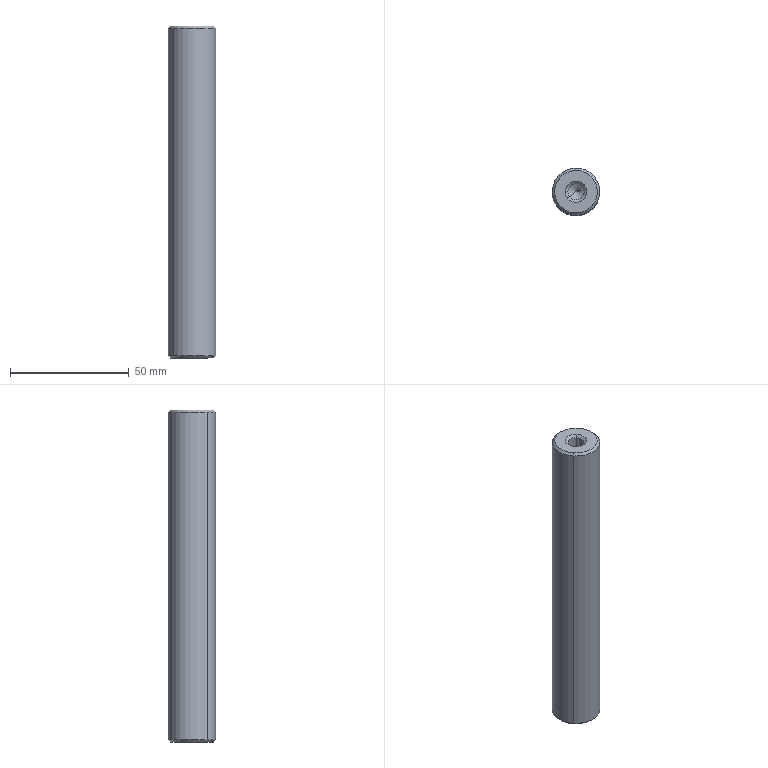Component | SolidWorks | Column-1 | 1 solid | 20 faces | box 20 x 20 x 140 mm | volume 42231 mm3 | cone 12 | cylinder 6 | plane 2 | commonest cylinder face diameters 6.8 x4 20 x2
STEP:
#1=COLOUR_RGB('',0.7922,0.8196,0.9333);
#2=FILL_AREA_STYLE_COLOUR('',#1);
#3=FILL_AREA_STYLE('',(#2));
#4=SURFACE_STYLE_FILL_AREA(#3);
#5=SURFACE_SIDE_STYLE('',(#4));
#6=SURFACE_STYLE_USAGE(.BOTH.,#5);
#7=PRESENTATION_STYLE_ASSIGNMENT((#6));
#8=CARTESIAN_POINT('',(-8.765,-5.597,0.3521));
#9=VERTEX_POINT('',#8);
#10=CARTESIAN_POINT('',(-8.558,-5.427,0.3521));
#11=VERTEX_POINT('',#10);
#12=CARTESIAN_POINT('',(-8.661,-5.512,0.3521));
#13=DIRECTION('',(0.,0.,-1.));
#14=DIRECTION('',(0.7722,0.6354,0.));
#15=AXIS2_PLACEMENT_3D('',#12,#13,#14);
#16=CIRCLE('',#15,0.1339);
#17=EDGE_CURVE('',#9,#11,#16,.T.);
#18=ORIENTED_EDGE('',*,*,#17,.F.);
#19=CARTESIAN_POINT('',(-8.799,-5.625,0.315));
#20=VERTEX_POINT('',#19);
#21=CARTESIAN_POINT('',(-8.799,-5.625,0.315));
#22=DIRECTION('',(-0.5915,-0.4867,-0.6428));
#23=VECTOR('',#22,39.37);
#24=LINE('',#21,#23);
#25=EDGE_CURVE('',#9,#20,#24,.T.);
#26=ORIENTED_EDGE('',*,*,#25,.T.);
#27=CARTESIAN_POINT('',(-8.524,-5.399,0.315));
#28=VERTEX_POINT('',#27);
#29=CARTESIAN_POINT('',(-8.661,-5.512,0.315));
#30=DIRECTION('',(0.,0.,-1.));
#31=DIRECTION('',(0.7722,0.6354,0.));
#32=AXIS2_PLACEMENT_3D('',#29,#30,#31);
#33=CIRCLE('',#32,0.1781);
#34=EDGE_CURVE('',#20,#28,#33,.T.);
#35=ORIENTED_EDGE('',*,*,#34,.T.);
#36=CARTESIAN_POINT('',(-8.524,-5.399,0.315));
#37=DIRECTION('',(0.5915,0.4867,-0.6428));
#38=VECTOR('',#37,39.37);
#39=LINE('',#36,#38);
#40=EDGE_CURVE('',#11,#28,#39,.T.);
#41=ORIENTED_EDGE('',*,*,#40,.F.);
#42=EDGE_LOOP('',(#18,#26,#35,#41));
#43=FACE_OUTER_BOUND('',#42,.T.);
#44=CARTESIAN_POINT('',(-8.661,-5.512,0.315));
#45=DIRECTION('',(0.,0.,-1.));
#46=DIRECTION('',(0.7722,0.6354,0.));
#47=AXIS2_PLACEMENT_3D('',#44,#45,#46);
#48=CONICAL_SURFACE('',#47,0.1781,0.8727);
#49=ADVANCED_FACE('',(#43),#48,.F.);
#50=CARTESIAN_POINT('',(-8.765,-5.597,1.191));
#51=VERTEX_POINT('',#50);
#52=CARTESIAN_POINT('',(-8.558,-5.427,1.191));
#53=VERTEX_POINT('',#52);
#54=CARTESIAN_POINT('',(-8.661,-5.512,1.191));
#55=DIRECTION('',(0.,0.,-1.));
#56=DIRECTION('',(0.7722,0.6354,0.));
#57=AXIS2_PLACEMENT_3D('',#54,#55,#56);
#58=CIRCLE('',#57,0.1339);
#59=EDGE_CURVE('',#51,#53,#58,.T.);
#60=ORIENTED_EDGE('',*,*,#59,.F.);
#61=CARTESIAN_POINT('',(-8.765,-5.597,0.315));
#62=DIRECTION('',(0.,0.,-1.));
#63=VECTOR('',#62,39.37);
#64=LINE('',#61,#63);
#65=EDGE_CURVE('',#51,#9,#64,.T.);
#66=ORIENTED_EDGE('',*,*,#65,.T.);
#67=ORIENTED_EDGE('',*,*,#17,.T.);
#68=CARTESIAN_POINT('',(-8.558,-5.427,0.315));
#69=DIRECTION('',(0.,0.,-1.));
#70=VECTOR('',#69,39.37);
#71=LINE('',#68,#70);
#72=EDGE_CURVE('',#53,#11,#71,.T.);
#73=ORIENTED_EDGE('',*,*,#72,.F.);
#74=EDGE_LOOP('',(#60,#66,#67,#73));
#75=FACE_OUTER_BOUND('',#74,.T.);
#76=CARTESIAN_POINT('',(-8.661,-5.512,0.315));
#77=DIRECTION('',(0.,0.,-1.));
#78=DIRECTION('',(0.7722,0.6354,0.));
#79=AXIS2_PLACEMENT_3D('',#76,#77,#78);
#80=CYLINDRICAL_SURFACE('',#79,0.1339);
#81=ADVANCED_FACE('',(#75),#80,.F.);
#82=CARTESIAN_POINT('',(-8.661,-5.512,1.271));
#83=VERTEX_POINT('',#82);
#84=CARTESIAN_POINT('',(-8.558,-5.427,1.191));
#85=DIRECTION('',(0.6619,0.5446,-0.515));
#86=VECTOR('',#85,39.37);
#87=LINE('',#84,#86);
#88=EDGE_CURVE('',#83,#53,#87,.T.);
#89=ORIENTED_EDGE('',*,*,#88,.F.);
#90=CARTESIAN_POINT('',(-8.765,-5.597,1.191));
#91=DIRECTION('',(-0.6619,-0.5446,-0.515));
#92=VECTOR('',#91,39.37);
#93=LINE('',#90,#92);
#94=EDGE_CURVE('',#83,#51,#93,.T.);
#95=ORIENTED_EDGE('',*,*,#94,.T.);
#96=ORIENTED_EDGE('',*,*,#59,.T.);
#97=EDGE_LOOP('',(#89,#95,#96));
#98=FACE_OUTER_BOUND('',#97,.T.);
#99=CARTESIAN_POINT('',(-8.661,-5.512,1.191));
#100=DIRECTION('',(0.,0.,-1.));
#101=DIRECTION('',(0.7722,0.6354,0.));
#102=AXIS2_PLACEMENT_3D('',#99,#100,#101);
#103=CONICAL_SURFACE('',#102,0.1339,1.03);
#104=ADVANCED_FACE('',(#98),#103,.F.);
#105=CARTESIAN_POINT('',(-8.558,-5.427,5.79));
#106=VERTEX_POINT('',#105);
#107=CARTESIAN_POINT('',(-8.765,-5.597,5.79));
#108=VERTEX_POINT('',#107);
#109=CARTESIAN_POINT('',(-8.661,-5.512,5.79));
#110=DIRECTION('',(-0.,-0.,1.));
#111=DIRECTION('',(-0.7722,-0.6354,0.));
#112=AXIS2_PLACEMENT_3D('',#109,#110,#111);
#113=CIRCLE('',#112,0.1339);
#114=EDGE_CURVE('',#106,#108,#113,.T.);
#115=ORIENTED_EDGE('',*,*,#114,.F.);
#116=CARTESIAN_POINT('',(-8.524,-5.399,5.827));
#117=VERTEX_POINT('',#116);
#118=CARTESIAN_POINT('',(-8.524,-5.399,5.827));
#119=DIRECTION('',(0.5915,0.4867,0.6428));
#120=VECTOR('',#119,39.37);
#121=LINE('',#118,#120);
#122=EDGE_CURVE('',#106,#117,#121,.T.);
#123=ORIENTED_EDGE('',*,*,#122,.T.);
#124=CARTESIAN_POINT('',(-8.799,-5.625,5.827));
#125=VERTEX_POINT('',#124);
#126=CARTESIAN_POINT('',(-8.661,-5.512,5.827));
#127=DIRECTION('',(-0.,-0.,1.));
#128=DIRECTION('',(-0.7722,-0.6354,0.));
#129=AXIS2_PLACEMENT_3D('',#126,#127,#128);
#130=CIRCLE('',#129,0.1781);
#131=EDGE_CURVE('',#117,#125,#130,.T.);
#132=ORIENTED_EDGE('',*,*,#131,.T.);
#133=CARTESIAN_POINT('',(-8.799,-5.625,5.827));
#134=DIRECTION('',(-0.5915,-0.4867,0.6428));
#135=VECTOR('',#134,39.37);
#136=LINE('',#133,#135);
#137=EDGE_CURVE('',#108,#125,#136,.T.);
#138=ORIENTED_EDGE('',*,*,#137,.F.);
#139=EDGE_LOOP('',(#115,#123,#132,#138));
#140=FACE_OUTER_BOUND('',#139,.T.);
#141=CARTESIAN_POINT('',(-8.661,-5.512,5.827));
#142=DIRECTION('',(-0.,-0.,1.));
#143=DIRECTION('',(-0.7722,-0.6354,0.));
#144=AXIS2_PLACEMENT_3D('',#141,#142,#143);
#145=CONICAL_SURFACE('',#144,0.1781,0.8727);
#146=ADVANCED_FACE('',(#140),#145,.F.);
#147=CARTESIAN_POINT('',(-8.558,-5.427,4.951));
#148=VERTEX_POINT('',#147);
#149=CARTESIAN_POINT('',(-8.765,-5.597,4.951));
#150=VERTEX_POINT('',#149);
#151=CARTESIAN_POINT('',(-8.661,-5.512,4.951));
#152=DIRECTION('',(-0.,-0.,1.));
#153=DIRECTION('',(-0.7722,-0.6354,0.));
#154=AXIS2_PLACEMENT_3D('',#151,#152,#153);
#155=CIRCLE('',#154,0.1339);
#156=EDGE_CURVE('',#148,#150,#155,.T.);
#157=ORIENTED_EDGE('',*,*,#156,.F.);
#158=CARTESIAN_POINT('',(-8.558,-5.427,5.827));
#159=DIRECTION('',(-0.,-0.,1.));
#160=VECTOR('',#159,39.37);
#161=LINE('',#158,#160);
#162=EDGE_CURVE('',#148,#106,#161,.T.);
#163=ORIENTED_EDGE('',*,*,#162,.T.);
#164=ORIENTED_EDGE('',*,*,#114,.T.);
#165=CARTESIAN_POINT('',(-8.765,-5.597,5.827));
#166=DIRECTION('',(-0.,-0.,1.));
#167=VECTOR('',#166,39.37);
#168=LINE('',#165,#167);
#169=EDGE_CURVE('',#150,#108,#168,.T.);
#170=ORIENTED_EDGE('',*,*,#169,.F.);
#171=EDGE_LOOP('',(#157,#163,#164,#170));
#172=FACE_OUTER_BOUND('',#171,.T.);
#173=CARTESIAN_POINT('',(-8.661,-5.512,5.827));
#174=DIRECTION('',(-0.,-0.,1.));
#175=DIRECTION('',(-0.7722,-0.6354,0.));
#176=AXIS2_PLACEMENT_3D('',#173,#174,#175);
#177=CYLINDRICAL_SURFACE('',#176,0.1339);
#178=ADVANCED_FACE('',(#172),#177,.F.);
#179=CARTESIAN_POINT('',(-8.661,-5.512,4.87));
#180=VERTEX_POINT('',#179);
#181=CARTESIAN_POINT('',(-8.765,-5.597,4.951));
#182=DIRECTION('',(-0.6619,-0.5446,0.515));
#183=VECTOR('',#182,39.37);
#184=LINE('',#181,#183);
#185=EDGE_CURVE('',#180,#150,#184,.T.);
#186=ORIENTED_EDGE('',*,*,#185,.F.);
#187=CARTESIAN_POINT('',(-8.558,-5.427,4.951));
#188=DIRECTION('',(0.6619,0.5446,0.515));
#189=VECTOR('',#188,39.37);
#190=LINE('',#187,#189);
#191=EDGE_CURVE('',#180,#148,#190,.T.);
#192=ORIENTED_EDGE('',*,*,#191,.T.);
#193=ORIENTED_EDGE('',*,*,#156,.T.);
#194=EDGE_LOOP('',(#186,#192,#193));
#195=FACE_OUTER_BOUND('',#194,.T.);
#196=CARTESIAN_POINT('',(-8.661,-5.512,4.951));
#197=DIRECTION('',(-0.,-0.,1.));
#198=DIRECTION('',(-0.7722,-0.6354,0.));
#199=AXIS2_PLACEMENT_3D('',#196,#197,#198);
#200=CONICAL_SURFACE('',#199,0.1339,1.03);
#201=ADVANCED_FACE('',(#195),#200,.F.);
#202=CARTESIAN_POINT('',(-8.935,-5.737,5.827));
#203=VERTEX_POINT('',#202);
#204=CARTESIAN_POINT('',(-8.388,-5.287,5.827));
#205=VERTEX_POINT('',#204);
#206=CARTESIAN_POINT('',(-8.661,-5.512,5.827));
#207=DIRECTION('',(-0.,-0.,1.));
#208=DIRECTION('',(-0.7722,-0.6354,-0.));
#209=AXIS2_PLACEMENT_3D('',#206,#207,#208);
#210=CIRCLE('',#209,0.3543);
#211=EDGE_CURVE('',#203,#205,#210,.T.);
#212=ORIENTED_EDGE('',*,*,#211,.F.);
#213=CARTESIAN_POINT('',(-8.965,-5.762,5.787));
#214=VERTEX_POINT('',#213);
#215=CARTESIAN_POINT('',(-8.935,-5.737,5.827));
#216=DIRECTION('',(-0.546,-0.4493,-0.7071));
#217=VECTOR('',#216,39.37);
#218=LINE('',#215,#217);
#219=EDGE_CURVE('',#203,#214,#218,.T.);
#220=ORIENTED_EDGE('',*,*,#219,.T.);
#221=CARTESIAN_POINT('',(-8.357,-5.262,5.787));
#222=VERTEX_POINT('',#221);
#223=CARTESIAN_POINT('',(-8.661,-5.512,5.787));
#224=DIRECTION('',(0.,0.,-1.));
#225=DIRECTION('',(-0.7722,-0.6354,-0.));
#226=AXIS2_PLACEMENT_3D('',#223,#224,#225);
#227=CIRCLE('',#226,0.3937);
#228=EDGE_CURVE('',#222,#214,#227,.T.);
#229=ORIENTED_EDGE('',*,*,#228,.F.);
#230=CARTESIAN_POINT('',(-8.388,-5.287,5.827));
#231=DIRECTION('',(0.546,0.4493,-0.7071));
#232=VECTOR('',#231,39.37);
#233=LINE('',#230,#232);
#234=EDGE_CURVE('',#205,#222,#233,.T.);
#235=ORIENTED_EDGE('',*,*,#234,.F.);
#236=EDGE_LOOP('',(#212,#220,#229,#235));
#237=FACE_OUTER_BOUND('',#236,.T.);
#238=CARTESIAN_POINT('',(-8.661,-5.512,5.827));
#239=DIRECTION('',(0.,0.,-1.));
#240=DIRECTION('',(0.7722,0.6354,0.));
#241=AXIS2_PLACEMENT_3D('',#238,#239,#240);
#242=CONICAL_SURFACE('',#241,0.3543,0.7854);
#243=ADVANCED_FACE('',(#237),#242,.T.);
#244=CARTESIAN_POINT('',(-8.388,-5.287,0.315));
#245=VERTEX_POINT('',#244);
#246=CARTESIAN_POINT('',(-8.935,-5.737,0.315));
#247=VERTEX_POINT('',#246);
#248=CARTESIAN_POINT('',(-8.661,-5.512,0.315));
#249=DIRECTION('',(0.,0.,-1.));
#250=DIRECTION('',(-0.7722,-0.6354,-0.));
#251=AXIS2_PLACEMENT_3D('',#248,#249,#250);
#252=CIRCLE('',#251,0.3543);
#253=EDGE_CURVE('',#245,#247,#252,.T.);
#254=ORIENTED_EDGE('',*,*,#253,.F.);
#255=CARTESIAN_POINT('',(-8.357,-5.262,0.3543));
#256=VERTEX_POINT('',#255);
#257=CARTESIAN_POINT('',(-8.357,-5.262,0.3543));
#258=DIRECTION('',(0.546,0.4493,0.7071));
#259=VECTOR('',#258,39.37);
#260=LINE('',#257,#259);
#261=EDGE_CURVE('',#245,#256,#260,.T.);
#262=ORIENTED_EDGE('',*,*,#261,.T.);
#263=CARTESIAN_POINT('',(-8.965,-5.762,0.3543));
#264=VERTEX_POINT('',#263);
#265=CARTESIAN_POINT('',(-8.661,-5.512,0.3543));
#266=DIRECTION('',(-0.,-0.,1.));
#267=DIRECTION('',(-0.7722,-0.6354,-0.));
#268=AXIS2_PLACEMENT_3D('',#265,#266,#267);
#269=CIRCLE('',#268,0.3937);
#270=EDGE_CURVE('',#264,#256,#269,.T.);
#271=ORIENTED_EDGE('',*,*,#270,.F.);
#272=CARTESIAN_POINT('',(-8.965,-5.762,0.3543));
#273=DIRECTION('',(-0.546,-0.4493,0.7071));
#274=VECTOR('',#273,39.37);
#275=LINE('',#272,#274);
#276=EDGE_CURVE('',#247,#264,#275,.T.);
#277=ORIENTED_EDGE('',*,*,#276,.F.);
#278=EDGE_LOOP('',(#254,#262,#271,#277));
#279=FACE_OUTER_BOUND('',#278,.T.);
#280=CARTESIAN_POINT('',(-8.661,-5.512,0.3543));
#281=DIRECTION('',(-0.,-0.,1.));
#282=DIRECTION('',(-0.7722,-0.6354,-0.));
#283=AXIS2_PLACEMENT_3D('',#280,#281,#282);
#284=CONICAL_SURFACE('',#283,0.3937,0.7854);
#285=ADVANCED_FACE('',(#279),#284,.T.);
#286=ORIENTED_EDGE('',*,*,#228,.T.);
#287=CARTESIAN_POINT('',(-8.965,-5.762,5.827));
#288=DIRECTION('',(0.,0.,-1.));
#289=VECTOR('',#288,39.37);
#290=LINE('',#287,#289);
#291=EDGE_CURVE('',#214,#264,#290,.T.);
#292=ORIENTED_EDGE('',*,*,#291,.T.);
#293=ORIENTED_EDGE('',*,*,#270,.T.);
#294=CARTESIAN_POINT('',(-8.357,-5.262,5.827));
#295=DIRECTION('',(0.,0.,-1.));
#296=VECTOR('',#295,39.37);
#297=LINE('',#294,#296);
#298=EDGE_CURVE('',#222,#256,#297,.T.);
#299=ORIENTED_EDGE('',*,*,#298,.F.);
#300=EDGE_LOOP('',(#286,#292,#293,#299));
#301=FACE_OUTER_BOUND('',#300,.T.);
#302=CARTESIAN_POINT('',(-8.661,-5.512,5.827));
#303=DIRECTION('',(0.,0.,-1.));
#304=DIRECTION('',(0.7722,0.6354,0.));
#305=AXIS2_PLACEMENT_3D('',#302,#303,#304);
#306=CYLINDRICAL_SURFACE('',#305,0.3937);
#307=ADVANCED_FACE('',(#301),#306,.T.);
#308=CARTESIAN_POINT('',(-8.661,-5.512,0.315));
#309=DIRECTION('',(0.,0.,-1.));
#310=DIRECTION('',(0.7722,0.6354,0.));
#311=AXIS2_PLACEMENT_3D('',#308,#309,#310);
#312=CIRCLE('',#311,0.1781);
#313=EDGE_CURVE('',#28,#20,#312,.T.);
#314=ORIENTED_EDGE('',*,*,#313,.F.);
#315=ORIENTED_EDGE('',*,*,#34,.F.);
#316=EDGE_LOOP('',(#314,#315));
#317=FACE_BOUND('',#316,.T.);
#318=CARTESIAN_POINT('',(-8.661,-5.512,0.315));
#319=DIRECTION('',(0.,0.,-1.));
#320=DIRECTION('',(-0.7722,-0.6354,-0.));
#321=AXIS2_PLACEMENT_3D('',#318,#319,#320);
#322=CIRCLE('',#321,0.3543);
#323=EDGE_CURVE('',#247,#245,#322,.T.);
#324=ORIENTED_EDGE('',*,*,#323,.T.);
#325=ORIENTED_EDGE('',*,*,#253,.T.);
#326=EDGE_LOOP('',(#324,#325));
#327=FACE_OUTER_BOUND('',#326,.T.);
#328=CARTESIAN_POINT('',(-8.661,-5.512,0.315));
#329=DIRECTION('',(-0.,-0.,1.));
#330=DIRECTION('',(-0.7722,-0.6354,-0.));
#331=AXIS2_PLACEMENT_3D('',#328,#329,#330);
#332=PLANE('',#331);
#333=ADVANCED_FACE('',(#317,#327),#332,.F.);
#334=CARTESIAN_POINT('',(-8.661,-5.512,5.827));
#335=DIRECTION('',(-0.,-0.,1.));
#336=DIRECTION('',(-0.7722,-0.6354,0.));
#337=AXIS2_PLACEMENT_3D('',#334,#335,#336);
#338=CIRCLE('',#337,0.1781);
#339=EDGE_CURVE('',#125,#117,#338,.T.);
#340=ORIENTED_EDGE('',*,*,#339,.F.);
#341=ORIENTED_EDGE('',*,*,#131,.F.);
#342=EDGE_LOOP('',(#340,#341));
#343=FACE_BOUND('',#342,.T.);
#344=CARTESIAN_POINT('',(-8.661,-5.512,5.827));
#345=DIRECTION('',(-0.,-0.,1.));
#346=DIRECTION('',(-0.7722,-0.6354,-0.));
#347=AXIS2_PLACEMENT_3D('',#344,#345,#346);
#348=CIRCLE('',#347,0.3543);
#349=EDGE_CURVE('',#205,#203,#348,.T.);
#350=ORIENTED_EDGE('',*,*,#349,.T.);
#351=ORIENTED_EDGE('',*,*,#211,.T.);
#352=EDGE_LOOP('',(#350,#351));
#353=FACE_OUTER_BOUND('',#352,.T.);
#354=CARTESIAN_POINT('',(-8.661,-5.512,5.827));
#355=DIRECTION('',(-0.,-0.,1.));
#356=DIRECTION('',(-0.7722,-0.6354,-0.));
#357=AXIS2_PLACEMENT_3D('',#354,#355,#356);
#358=PLANE('',#357);
#359=ADVANCED_FACE('',(#343,#353),#358,.T.);
#360=ORIENTED_EDGE('',*,*,#291,.F.);
#361=CARTESIAN_POINT('',(-8.661,-5.512,5.787));
#362=DIRECTION('',(0.,0.,-1.));
#363=DIRECTION('',(-0.7722,-0.6354,-0.));
#364=AXIS2_PLACEMENT_3D('',#361,#362,#363);
#365=CIRCLE('',#364,0.3937);
#366=EDGE_CURVE('',#214,#222,#365,.T.);
#367=ORIENTED_EDGE('',*,*,#366,.T.);
#368=ORIENTED_EDGE('',*,*,#298,.T.);
#369=CARTESIAN_POINT('',(-8.661,-5.512,0.3543));
#370=DIRECTION('',(-0.,-0.,1.));
#371=DIRECTION('',(-0.7722,-0.6354,-0.));
#372=AXIS2_PLACEMENT_3D('',#369,#370,#371);
#373=CIRCLE('',#372,0.3937);
#374=EDGE_CURVE('',#256,#264,#373,.T.);
#375=ORIENTED_EDGE('',*,*,#374,.T.);
#376=EDGE_LOOP('',(#360,#367,#368,#375));
#377=FACE_OUTER_BOUND('',#376,.T.);
#378=CARTESIAN_POINT('',(-8.661,-5.512,5.827));
#379=DIRECTION('',(0.,0.,-1.));
#380=DIRECTION('',(0.7722,0.6354,0.));
#381=AXIS2_PLACEMENT_3D('',#378,#379,#380);
#382=CYLINDRICAL_SURFACE('',#381,0.3937);
#383=ADVANCED_FACE('',(#377),#382,.T.);
#384=ORIENTED_EDGE('',*,*,#261,.F.);
#385=ORIENTED_EDGE('',*,*,#323,.F.);
#386=ORIENTED_EDGE('',*,*,#276,.T.);
#387=ORIENTED_EDGE('',*,*,#374,.F.);
#388=EDGE_LOOP('',(#384,#385,#386,#387));
#389=FACE_OUTER_BOUND('',#388,.T.);
#390=CARTESIAN_POINT('',(-8.661,-5.512,0.3543));
#391=DIRECTION('',(-0.,-0.,1.));
#392=DIRECTION('',(-0.7722,-0.6354,-0.));
#393=AXIS2_PLACEMENT_3D('',#390,#391,#392);
#394=CONICAL_SURFACE('',#393,0.3937,0.7854);
#395=ADVANCED_FACE('',(#389),#394,.T.);
#396=ORIENTED_EDGE('',*,*,#219,.F.);
#397=ORIENTED_EDGE('',*,*,#349,.F.);
#398=ORIENTED_EDGE('',*,*,#234,.T.);
#399=ORIENTED_EDGE('',*,*,#366,.F.);
#400=EDGE_LOOP('',(#396,#397,#398,#399));
#401=FACE_OUTER_BOUND('',#400,.T.);
#402=CARTESIAN_POINT('',(-8.661,-5.512,5.827));
#403=DIRECTION('',(0.,0.,-1.));
#404=DIRECTION('',(0.7722,0.6354,0.));
#405=AXIS2_PLACEMENT_3D('',#402,#403,#404);
#406=CONICAL_SURFACE('',#405,0.3543,0.7854);
#407=ADVANCED_FACE('',(#401),#406,.T.);
#408=ORIENTED_EDGE('',*,*,#191,.F.);
#409=ORIENTED_EDGE('',*,*,#185,.T.);
#410=CARTESIAN_POINT('',(-8.661,-5.512,4.951));
#411=DIRECTION('',(-0.,-0.,1.));
#412=DIRECTION('',(-0.7722,-0.6354,0.));
#413=AXIS2_PLACEMENT_3D('',#410,#411,#412);
#414=CIRCLE('',#413,0.1339);
#415=EDGE_CURVE('',#150,#148,#414,.T.);
#416=ORIENTED_EDGE('',*,*,#415,.T.);
#417=EDGE_LOOP('',(#408,#409,#416));
#418=FACE_OUTER_BOUND('',#417,.T.);
#419=CARTESIAN_POINT('',(-8.661,-5.512,4.951));
#420=DIRECTION('',(-0.,-0.,1.));
#421=DIRECTION('',(-0.7722,-0.6354,0.));
#422=AXIS2_PLACEMENT_3D('',#419,#420,#421);
#423=CONICAL_SURFACE('',#422,0.1339,1.03);
#424=ADVANCED_FACE('',(#418),#423,.F.);
#425=ORIENTED_EDGE('',*,*,#162,.F.);
#426=ORIENTED_EDGE('',*,*,#415,.F.);
#427=ORIENTED_EDGE('',*,*,#169,.T.);
#428=CARTESIAN_POINT('',(-8.661,-5.512,5.79));
#429=DIRECTION('',(-0.,-0.,1.));
#430=DIRECTION('',(-0.7722,-0.6354,0.));
#431=AXIS2_PLACEMENT_3D('',#428,#429,#430);
#432=CIRCLE('',#431,0.1339);
#433=EDGE_CURVE('',#108,#106,#432,.T.);
#434=ORIENTED_EDGE('',*,*,#433,.T.);
#435=EDGE_LOOP('',(#425,#426,#427,#434));
#436=FACE_OUTER_BOUND('',#435,.T.);
#437=CARTESIAN_POINT('',(-8.661,-5.512,5.827));
#438=DIRECTION('',(-0.,-0.,1.));
#439=DIRECTION('',(-0.7722,-0.6354,0.));
#440=AXIS2_PLACEMENT_3D('',#437,#438,#439);
#441=CYLINDRICAL_SURFACE('',#440,0.1339);
#442=ADVANCED_FACE('',(#436),#441,.F.);
#443=ORIENTED_EDGE('',*,*,#122,.F.);
#444=ORIENTED_EDGE('',*,*,#433,.F.);
#445=ORIENTED_EDGE('',*,*,#137,.T.);
#446=ORIENTED_EDGE('',*,*,#339,.T.);
#447=EDGE_LOOP('',(#443,#444,#445,#446));
#448=FACE_OUTER_BOUND('',#447,.T.);
#449=CARTESIAN_POINT('',(-8.661,-5.512,5.827));
#450=DIRECTION('',(-0.,-0.,1.));
#451=DIRECTION('',(-0.7722,-0.6354,0.));
#452=AXIS2_PLACEMENT_3D('',#449,#450,#451);
#453=CONICAL_SURFACE('',#452,0.1781,0.8727);
#454=ADVANCED_FACE('',(#448),#453,.F.);
#455=ORIENTED_EDGE('',*,*,#94,.F.);
#456=ORIENTED_EDGE('',*,*,#88,.T.);
#457=CARTESIAN_POINT('',(-8.661,-5.512,1.191));
#458=DIRECTION('',(0.,0.,-1.));
#459=DIRECTION('',(0.7722,0.6354,0.));
#460=AXIS2_PLACEMENT_3D('',#457,#458,#459);
#461=CIRCLE('',#460,0.1339);
#462=EDGE_CURVE('',#53,#51,#461,.T.);
#463=ORIENTED_EDGE('',*,*,#462,.T.);
#464=EDGE_LOOP('',(#455,#456,#463));
#465=FACE_OUTER_BOUND('',#464,.T.);
#466=CARTESIAN_POINT('',(-8.661,-5.512,1.191));
#467=DIRECTION('',(0.,0.,-1.));
#468=DIRECTION('',(0.7722,0.6354,0.));
#469=AXIS2_PLACEMENT_3D('',#466,#467,#468);
#470=CONICAL_SURFACE('',#469,0.1339,1.03);
#471=ADVANCED_FACE('',(#465),#470,.F.);
#472=ORIENTED_EDGE('',*,*,#65,.F.);
#473=ORIENTED_EDGE('',*,*,#462,.F.);
#474=ORIENTED_EDGE('',*,*,#72,.T.);
#475=CARTESIAN_POINT('',(-8.661,-5.512,0.3521));
#476=DIRECTION('',(0.,0.,-1.));
#477=DIRECTION('',(0.7722,0.6354,0.));
#478=AXIS2_PLACEMENT_3D('',#475,#476,#477);
#479=CIRCLE('',#478,0.1339);
#480=EDGE_CURVE('',#11,#9,#479,.T.);
#481=ORIENTED_EDGE('',*,*,#480,.T.);
#482=EDGE_LOOP('',(#472,#473,#474,#481));
#483=FACE_OUTER_BOUND('',#482,.T.);
#484=CARTESIAN_POINT('',(-8.661,-5.512,0.315));
#485=DIRECTION('',(0.,0.,-1.));
#486=DIRECTION('',(0.7722,0.6354,0.));
#487=AXIS2_PLACEMENT_3D('',#484,#485,#486);
#488=CYLINDRICAL_SURFACE('',#487,0.1339);
#489=ADVANCED_FACE('',(#483),#488,.F.);
#490=ORIENTED_EDGE('',*,*,#25,.F.);
#491=ORIENTED_EDGE('',*,*,#480,.F.);
#492=ORIENTED_EDGE('',*,*,#40,.T.);
#493=ORIENTED_EDGE('',*,*,#313,.T.);
#494=EDGE_LOOP('',(#490,#491,#492,#493));
#495=FACE_OUTER_BOUND('',#494,.T.);
#496=CARTESIAN_POINT('',(-8.661,-5.512,0.315));
#497=DIRECTION('',(0.,0.,-1.));
#498=DIRECTION('',(0.7722,0.6354,0.));
#499=AXIS2_PLACEMENT_3D('',#496,#497,#498);
#500=CONICAL_SURFACE('',#499,0.1781,0.8727);
#501=ADVANCED_FACE('',(#495),#500,.F.);
#502=CLOSED_SHELL('',(#49,#81,#104,#146,#178,#201,#243,#285,#307,#333,#359,#383,#395,#407,#424,#442,#454,#471,#489,#501));
#503=MANIFOLD_SOLID_BREP('',#502);
#504=STYLED_ITEM('',(#7),#503);
#505=PRESENTATION_LAYER_ASSIGNMENT('','',(#504));
#506=CARTESIAN_POINT('',(0.,0.,0.));
#507=DIRECTION('',(0.,0.,1.));
#508=DIRECTION('',(1.,0.,0.));
#509=AXIS2_PLACEMENT_3D('',#506,#507,#508);
#510=(LENGTH_UNIT()NAMED_UNIT(*)SI_UNIT($,.METRE.));
#511=LENGTH_MEASURE_WITH_UNIT(LENGTH_MEASURE(0.0254),#510);
#512=DIMENSIONAL_EXPONENTS(1.,0.,0.,0.,0.,0.,0.);
#513=(CONVERSION_BASED_UNIT('',#511)LENGTH_UNIT()NAMED_UNIT(#512));
#514=UNCERTAINTY_MEASURE_WITH_UNIT(LENGTH_MEASURE(0.00001),#513,'','');
#515=(NAMED_UNIT(*)PLANE_ANGLE_UNIT()SI_UNIT($,.RADIAN.));
#516=(NAMED_UNIT(*)SI_UNIT($,.STERADIAN.)SOLID_ANGLE_UNIT());
#517=(GEOMETRIC_REPRESENTATION_CONTEXT(3)GLOBAL_UNCERTAINTY_ASSIGNED_CONTEXT((#514))GLOBAL_UNIT_ASSIGNED_CONTEXT((#513,#515,#516))REPRESENTATION_CONTEXT('',''));
#518=ADVANCED_BREP_SHAPE_REPRESENTATION('',(#503,#509),#517);
#519=(LENGTH_UNIT()NAMED_UNIT(*)SI_UNIT($,.METRE.));
#520=LENGTH_MEASURE_WITH_UNIT(LENGTH_MEASURE(0.0254),#519);
#521=DIMENSIONAL_EXPONENTS(1.,0.,0.,0.,0.,0.,0.);
#522=(CONVERSION_BASED_UNIT('',#520)LENGTH_UNIT()NAMED_UNIT(#521));
#523=UNCERTAINTY_MEASURE_WITH_UNIT(LENGTH_MEASURE(0.00001),#522,'','');
#524=(NAMED_UNIT(*)PLANE_ANGLE_UNIT()SI_UNIT($,.RADIAN.));
#525=(NAMED_UNIT(*)SI_UNIT($,.STERADIAN.)SOLID_ANGLE_UNIT());
#526=(GEOMETRIC_REPRESENTATION_CONTEXT(3)GLOBAL_UNCERTAINTY_ASSIGNED_CONTEXT((#523))GLOBAL_UNIT_ASSIGNED_CONTEXT((#522,#524,#525))REPRESENTATION_CONTEXT('',''));
#527=MECHANICAL_DESIGN_GEOMETRIC_PRESENTATION_REPRESENTATION('',(#504),#526);